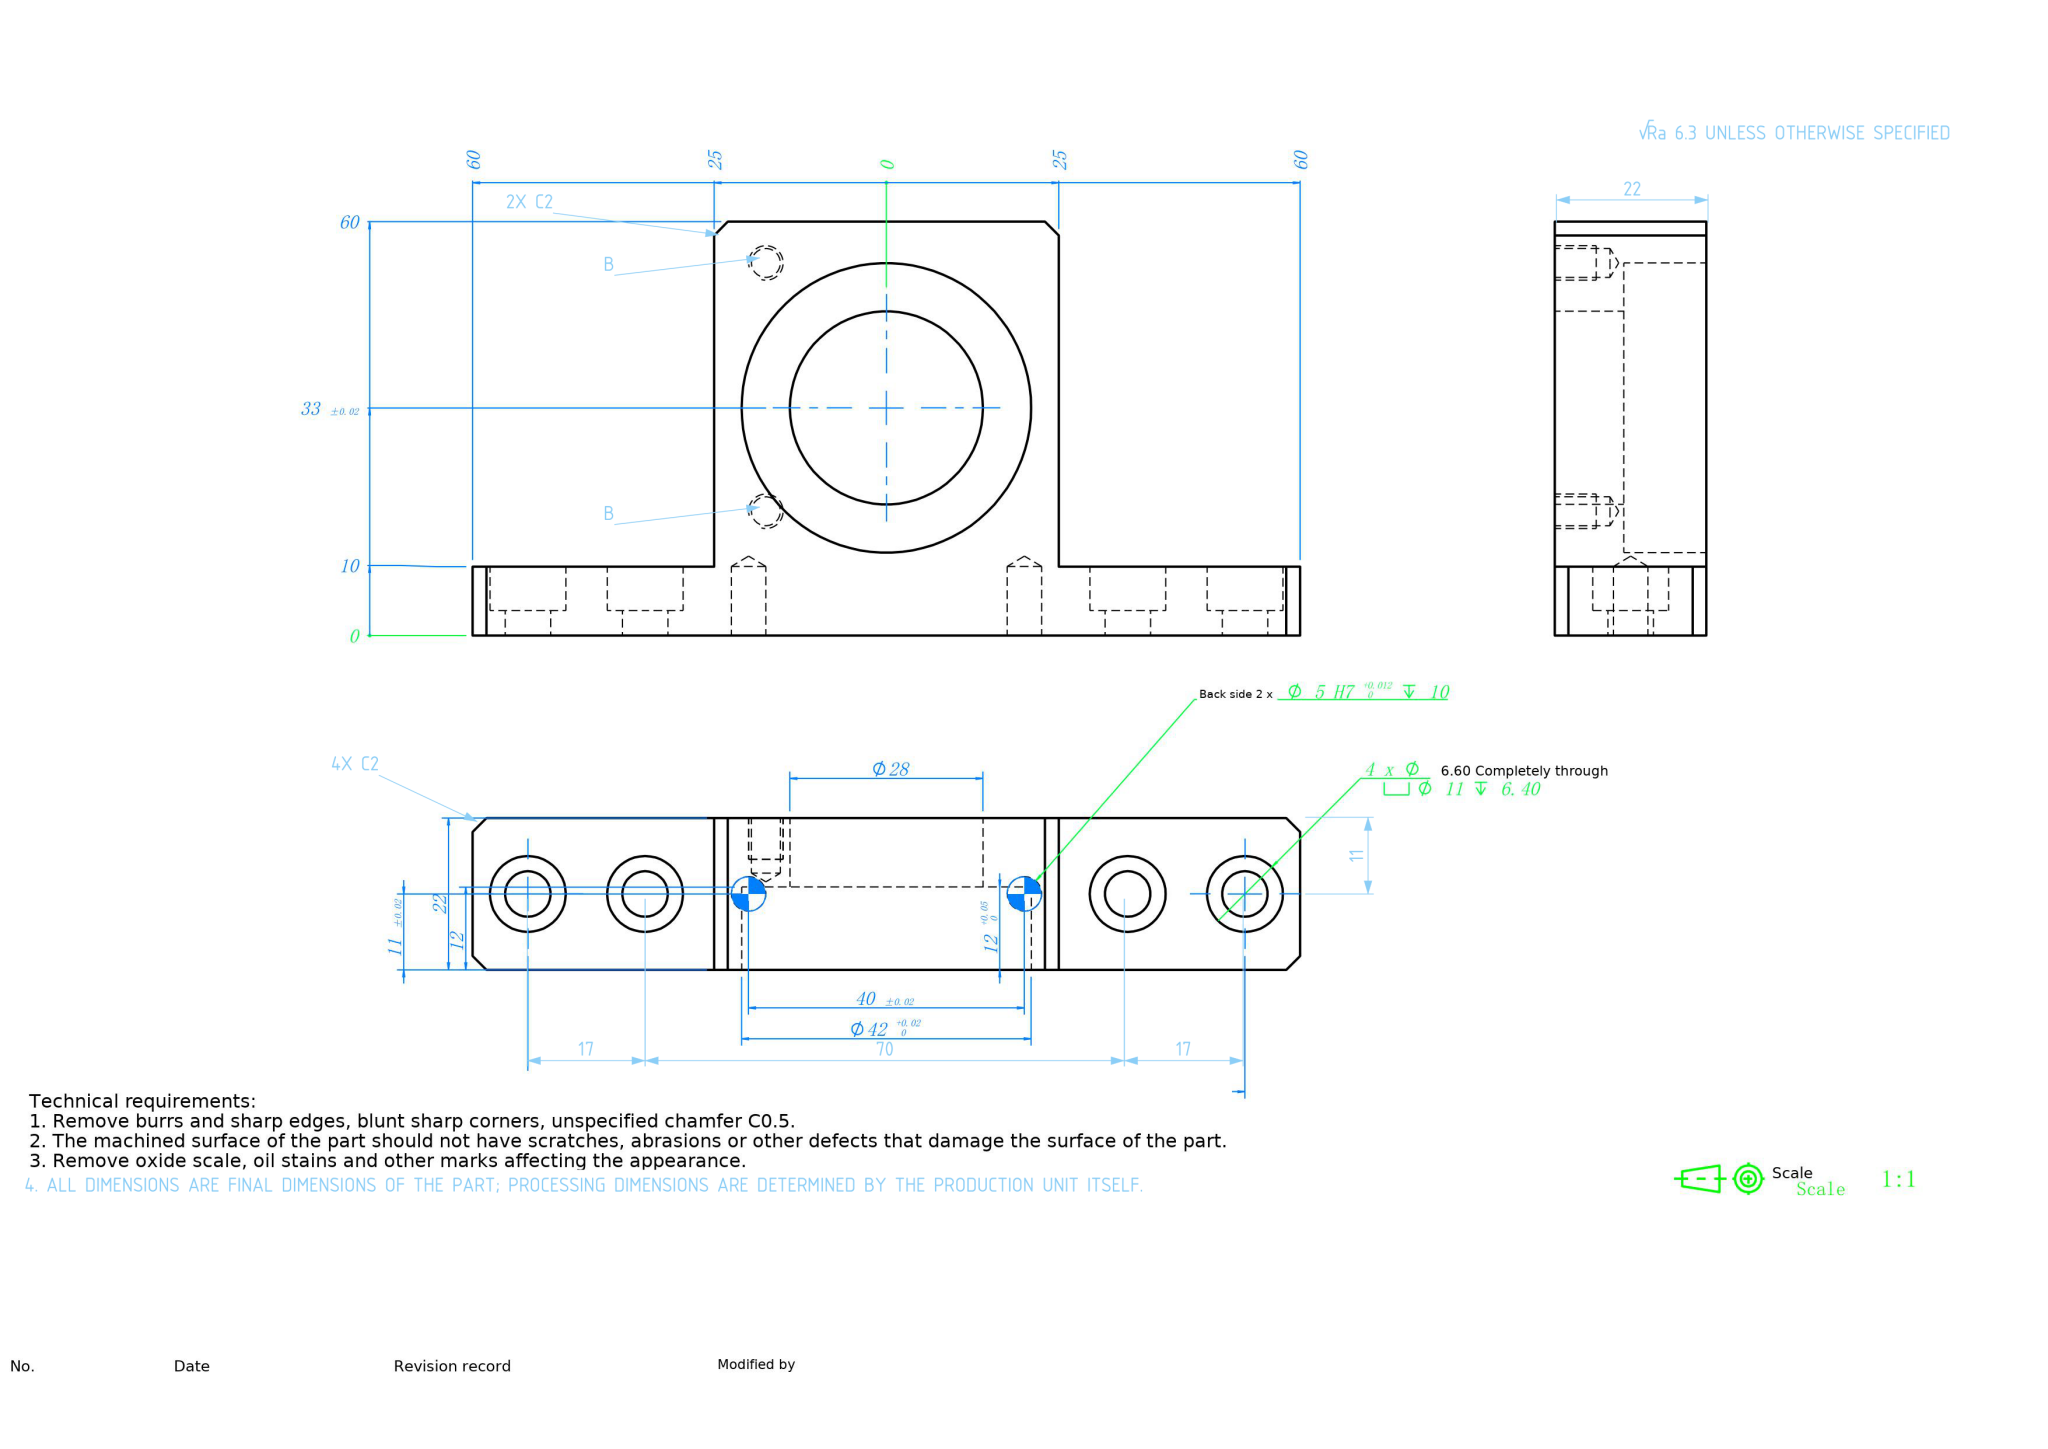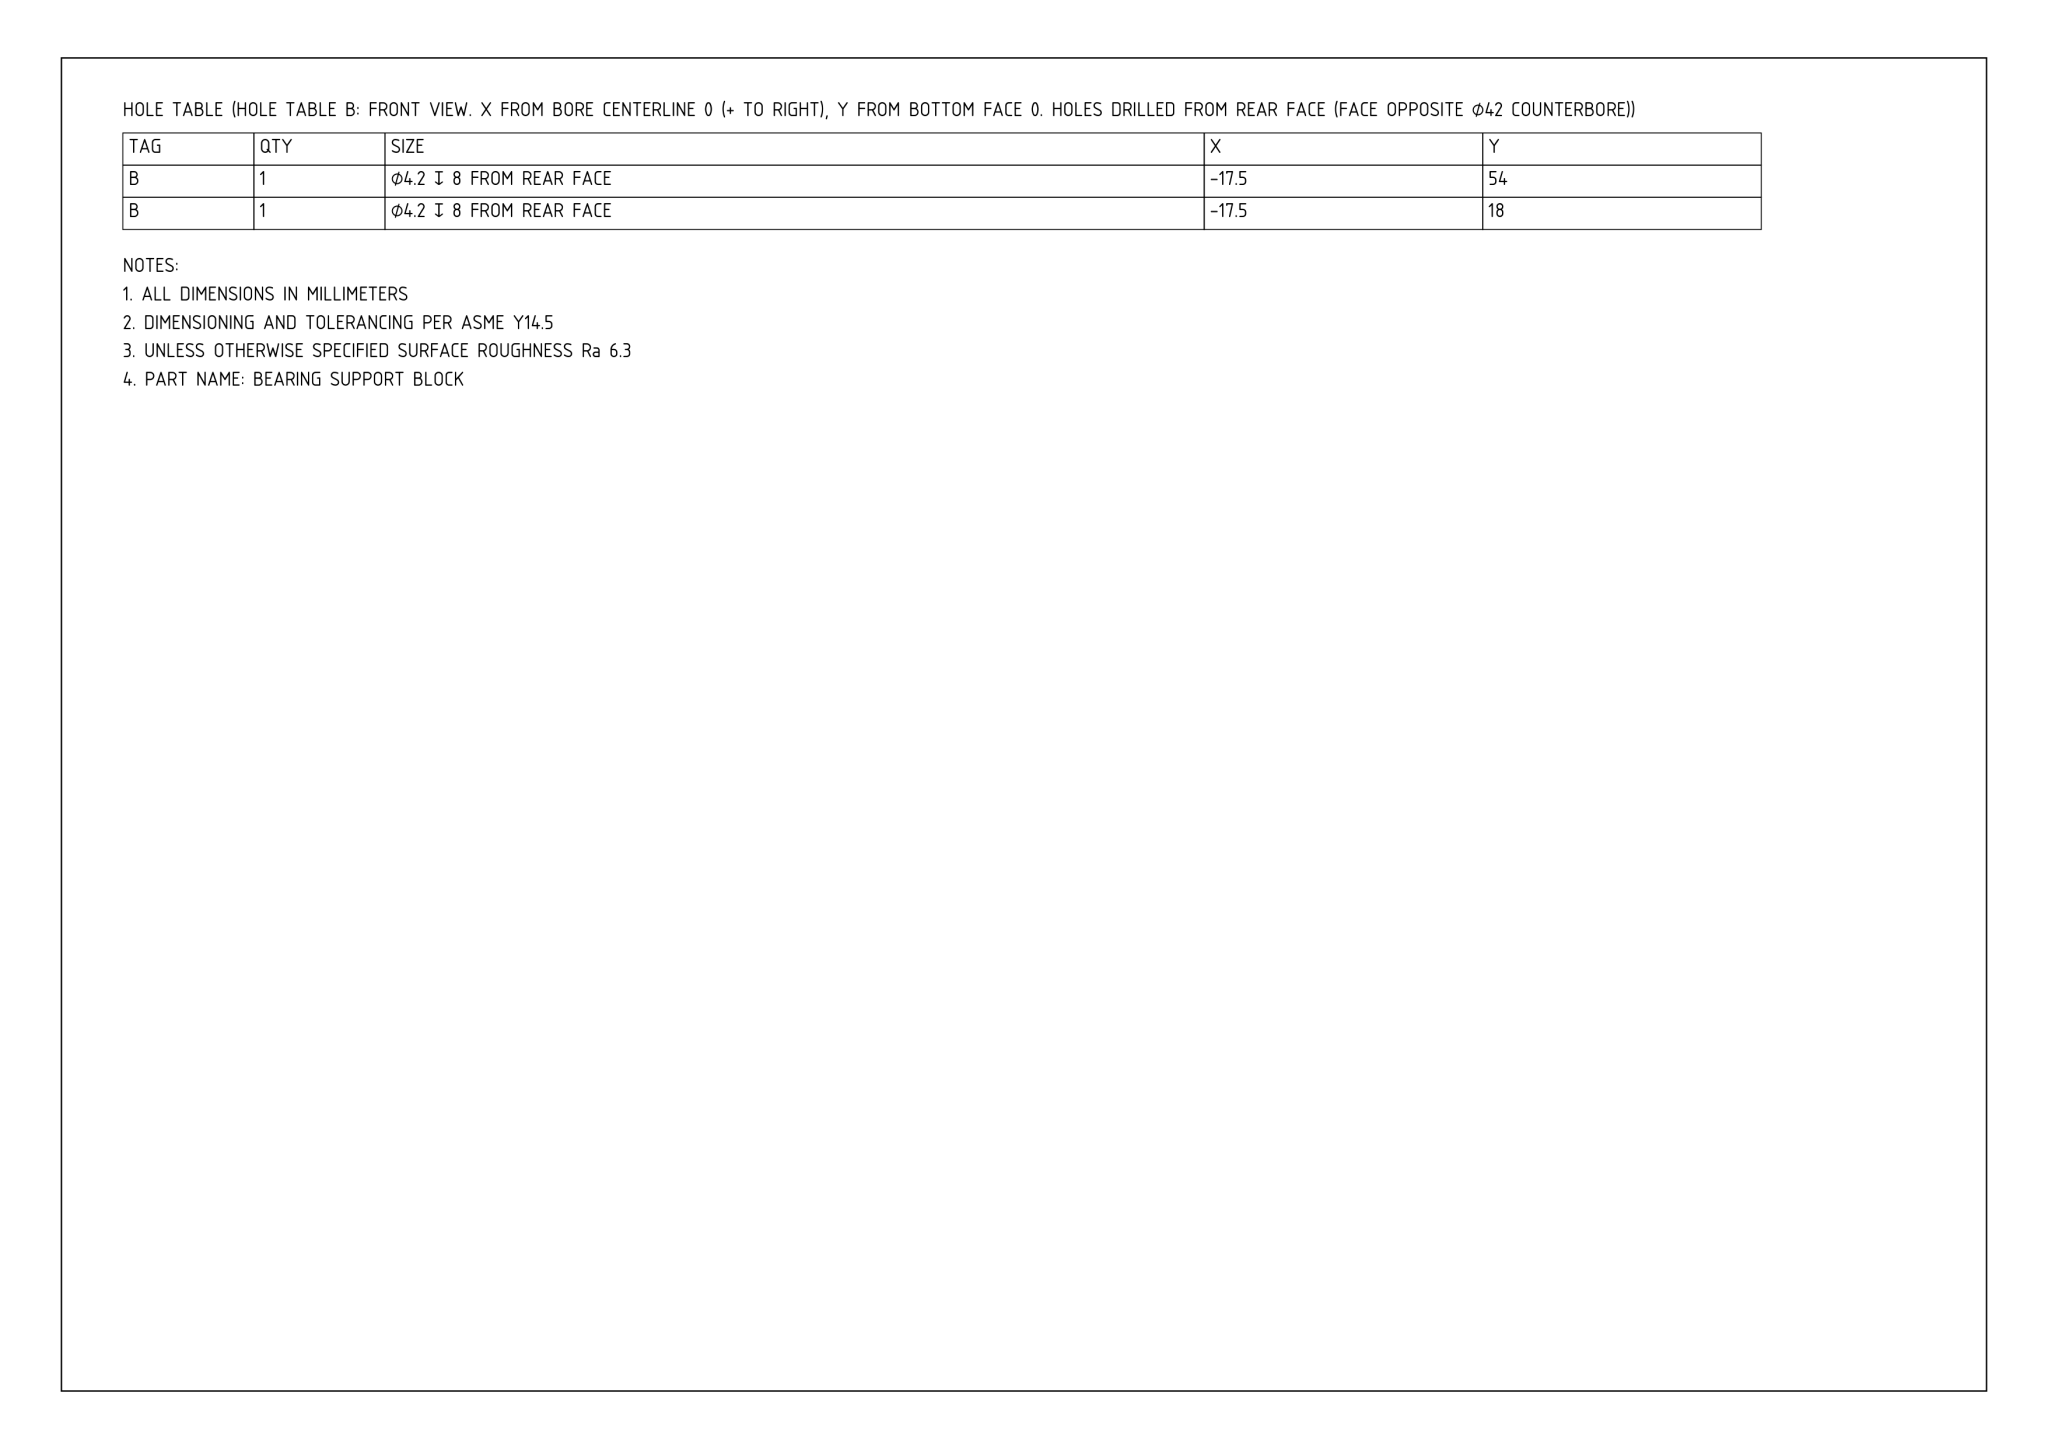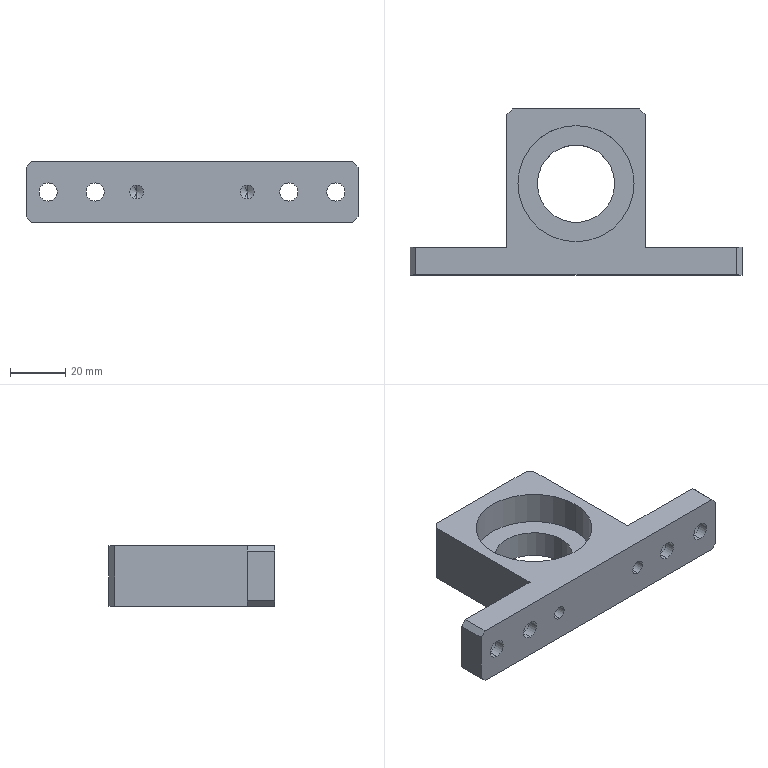Part | NX | mm | 1 solid | 57 faces | box 120 x 60 x 22 mm | volume 54878 mm3 | cylinder 28 | plane 21 | cone 8 | commonest cylinder face diameters 11 x8 6.6 x8 4.2 x4 5 x4 42 x2 28 x2